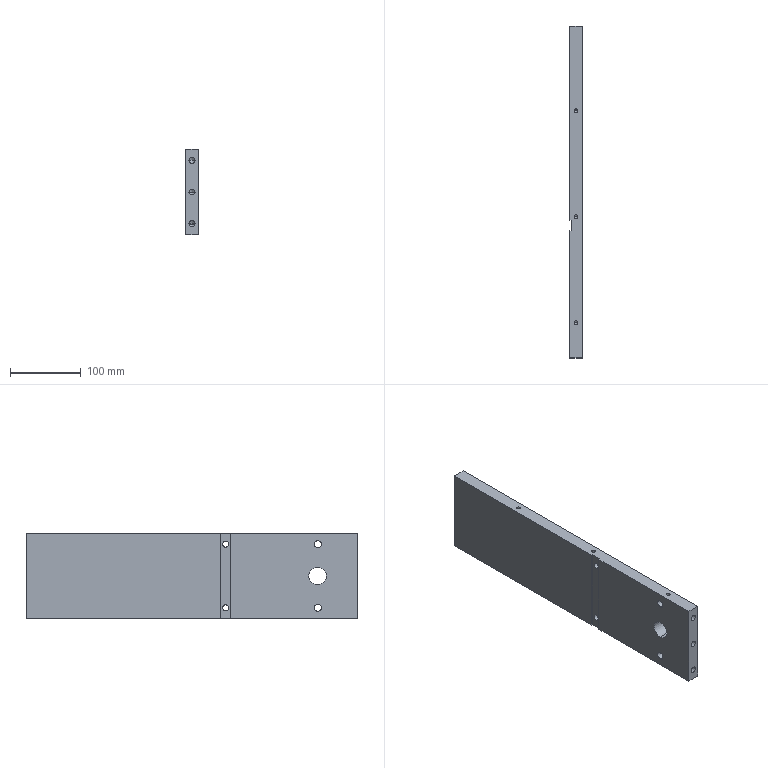Component | SolidWorks | ZL-11-05LargeUprightPlate2-1 | 1 solid | 68 faces | box 18 x 470 x 121 mm | volume 996568 mm3 | cylinder 34 | cone 24 | plane 10 | commonest cylinder face diameters 8.5 x16 5 x12 10.2 x4 25 x2
build123d program:
from build123d import *

# Parameters (mm, degrees)
SKETCH1_W                   = 121
SKETCH1_H                   = 470
EXTRUDE1_DEPTH              = 18
F_25_0_25_DIAMETER_HOLE1_D  = 25
M12_TAPPED_HOLE1_D          = 10.2
SKETCH6_W                   = 121
SKETCH6_H                   = 15
CUT_EXTRUDE1_DEPTH          = 2
F_8_5_8_5_DIAMETER_HOLE1_D  = 8.5
M10_TAPPED_HOLE2_AT_2_COUNT = 2
M10_TAPPED_HOLE2_AT_2_PITCH = 45
M10_TAPPED_HOLE2_AT_3_COUNT = 2
M10_TAPPED_HOLE2_AT_3_PITCH = 45
LPATTERN1_COUNT             = 3
LPATTERN1_PITCH             = 150


with BuildPart() as part:
    # Sketch1 → Extrude1 (new body)
    with BuildSketch(Plane.XY):
        Rectangle(SKETCH1_W, SKETCH1_H)
    extrude(amount=EXTRUDE1_DEPTH)

    # 25.0 _25_ Diameter Hole1 (through all)
    with Locations(Plane(origin=(0, 178, 0), x_dir=(-1, 0, 0), z_dir=(0, 0, -1))):
        with Locations((0, 0)):
            Hole(F_25_0_25_DIAMETER_HOLE1_D / 2)

    # M12 Tapped Hole1 (through all)
    with Locations(Plane(origin=(45, 178, 0), x_dir=(-1, 0, 0), z_dir=(0, 0, -1))):
        with Locations((0, 0), (90, 0)):
            Hole(M12_TAPPED_HOLE1_D / 2)

    # Sketch6 → Cut-Extrude1 (cut)
    with BuildSketch(Plane(origin=(0, 0, 0), x_dir=(-1, 0, 0), z_dir=(0, 0, -1))):
        with Locations((0, 47.5)):
            Rectangle(SKETCH6_W, SKETCH6_H)
    extrude(amount=-CUT_EXTRUDE1_DEPTH, mode=Mode.SUBTRACT)

    # 8.5 _8.5_ Diameter Hole1 (through all)
    with Locations(Plane(origin=(0, 0, 2), x_dir=(-1, 0, 0), z_dir=(0, 0, -1))):
        with Locations((45, 47.5), (-45, 47.5)):
            Hole(F_8_5_8_5_DIAMETER_HOLE1_D / 2)

    # Sketch12 → M10 Tapped Hole2 (revolve, cut)
    with BuildSketch(Plane(origin=(0, 235, 9), x_dir=(0, 0, 1), z_dir=(1, 0, 0))):
        Polygon((0, 0), (0, 27.054), (4.25, 24.5), (4.25, 0), align=None)
    m10_tapped_hole2 = revolve(axis=Axis((0, 241.35, 9), (0, -1, 0)), mode=Mode.SUBTRACT)

    # M10 Tapped Hole2 at 2: M10 Tapped Hole2 ×2
    with Locations(*[(-i * M10_TAPPED_HOLE2_AT_2_PITCH, 0, 0) for i in range(1, M10_TAPPED_HOLE2_AT_2_COUNT)]):
        add(m10_tapped_hole2, mode=Mode.SUBTRACT)

    # M10 Tapped Hole2 at 3: M10 Tapped Hole2 ×2
    with Locations(*[(i * M10_TAPPED_HOLE2_AT_3_PITCH, 0, 0) for i in range(1, M10_TAPPED_HOLE2_AT_3_COUNT)]):
        add(m10_tapped_hole2, mode=Mode.SUBTRACT)

    # Sketch13 → M6 Tapped Hole1 (revolve, cut)
    with BuildSketch(Plane(origin=(-60.5, 185, 9), x_dir=(0, 0, 1), z_dir=(0, 1, 0))):
        Polygon((0, 0), (0, 11.502), (2.5, 10), (2.5, 0), align=None)
    m6_tapped_hole1 = revolve(axis=Axis((-66.85, 185, 9), (1, 0, 0)), mode=Mode.SUBTRACT)

    # LPattern1: M6 Tapped Hole1 ×3
    with Locations(*[(0, -i * LPATTERN1_PITCH, 0) for i in range(1, LPATTERN1_COUNT)]):
        add(m6_tapped_hole1, mode=Mode.SUBTRACT)

    # Mirror1: M6 Tapped Hole1 across plane
    add(m6_tapped_hole1.mirror(Plane(origin=(0, 0, 0), x_dir=(0, 0, 1), z_dir=(1, 0, 0))), mode=Mode.SUBTRACT)

    # Mirror1 copy 1 sketch → Mirror1 copy 1 (revolve, cut)
    with BuildSketch(Plane(origin=(60.5, 35, 9), x_dir=(0, 0, 1), z_dir=(0, 1, 0))):
        Polygon((0, 0), (0, -11.502), (2.5, -10), (2.5, 0), align=None)
    revolve(axis=Axis((66.85, 35, 9), (1, 0, 0)), mode=Mode.SUBTRACT)

    # Mirror1 copy 2 sketch → Mirror1 copy 2 (revolve, cut)
    with BuildSketch(Plane(origin=(60.5, -115, 9), x_dir=(0, 0, 1), z_dir=(0, 1, 0))):
        Polygon((0, 0), (0, -11.502), (2.5, -10), (2.5, 0), align=None)
    revolve(axis=Axis((66.85, -115, 9), (1, 0, 0)), mode=Mode.SUBTRACT)

    # Mirror2: M10 Tapped Hole2 across plane
    add(m10_tapped_hole2.mirror(Plane.ZX), mode=Mode.SUBTRACT)

    # Mirror2 copy 1 sketch → Mirror2 copy 1 (revolve, cut)
    with BuildSketch(Plane(origin=(-45, -235, 9), x_dir=(0, 0, 1), z_dir=(1, 0, 0))):
        Polygon((0, 0), (0, -27.054), (4.25, -24.5), (4.25, 0), align=None)
    revolve(axis=Axis((-45, -241.35, 9), (0, -1, 0)), mode=Mode.SUBTRACT)

    # Mirror2 copy 2 sketch → Mirror2 copy 2 (revolve, cut)
    with BuildSketch(Plane(origin=(45, -235, 9), x_dir=(0, 0, 1), z_dir=(1, 0, 0))):
        Polygon((0, 0), (0, -27.054), (4.25, -24.5), (4.25, 0), align=None)
    revolve(axis=Axis((45, -241.35, 9), (0, -1, 0)), mode=Mode.SUBTRACT)


solid = part.part

# Placed as in the assembly
solid = solid.moved(Location((175.552, 289.22, 0), (180, 90, 0)))